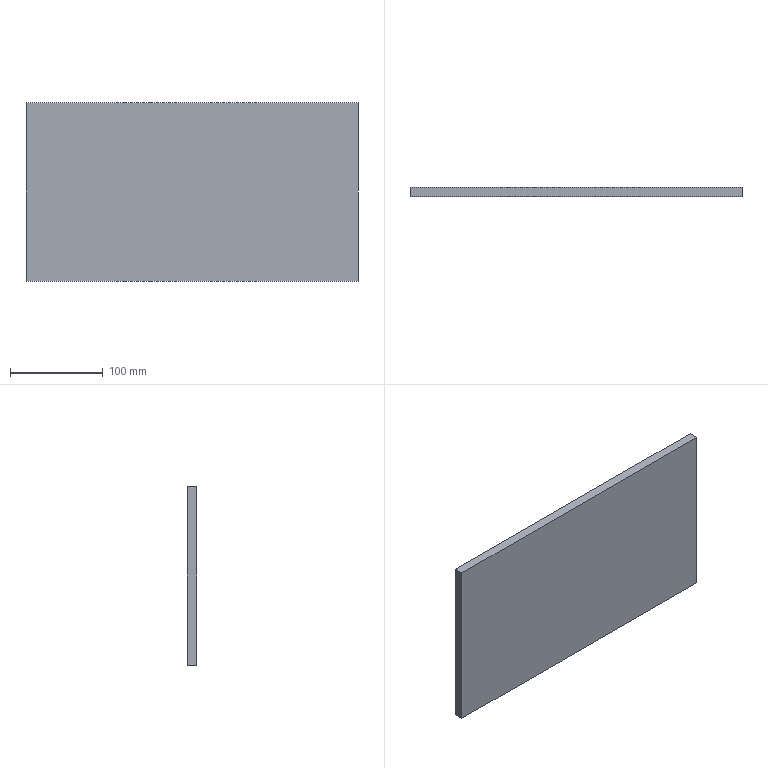Component | SolidWorks | ColumnRibPlate-1 | 1 solid | 6 faces | box 358 x 10 x 192 mm | volume 687360 mm3 | plane 6 | material Plain Carbon Steel
STEP:
#1=COLOUR_RGB('',0.7922,0.8196,0.9333);
#2=FILL_AREA_STYLE_COLOUR('',#1);
#3=FILL_AREA_STYLE('',(#2));
#4=SURFACE_STYLE_FILL_AREA(#3);
#5=SURFACE_SIDE_STYLE('',(#4));
#6=SURFACE_STYLE_USAGE(.BOTH.,#5);
#7=PRESENTATION_STYLE_ASSIGNMENT((#6));
#8=CARTESIAN_POINT('',(33.226,97.705,80.917));
#9=VERTEX_POINT('',#8);
#10=CARTESIAN_POINT('',(33.226,97.705,73.358));
#11=VERTEX_POINT('',#10);
#12=CARTESIAN_POINT('',(33.226,97.705,73.358));
#13=DIRECTION('',(-0.,0.,-1.));
#14=VECTOR('',#13,39.37);
#15=LINE('',#12,#14);
#16=EDGE_CURVE('',#9,#11,#15,.T.);
#17=ORIENTED_EDGE('',*,*,#16,.F.);
#18=CARTESIAN_POINT('',(33.226,97.311,80.917));
#19=VERTEX_POINT('',#18);
#20=CARTESIAN_POINT('',(33.226,97.311,80.917));
#21=DIRECTION('',(0.,1.,0.));
#22=VECTOR('',#21,39.37);
#23=LINE('',#20,#22);
#24=EDGE_CURVE('',#19,#9,#23,.T.);
#25=ORIENTED_EDGE('',*,*,#24,.F.);
#26=CARTESIAN_POINT('',(33.226,97.311,73.358));
#27=VERTEX_POINT('',#26);
#28=CARTESIAN_POINT('',(33.226,97.311,73.358));
#29=DIRECTION('',(-0.,0.,-1.));
#30=VECTOR('',#29,39.37);
#31=LINE('',#28,#30);
#32=EDGE_CURVE('',#19,#27,#31,.T.);
#33=ORIENTED_EDGE('',*,*,#32,.T.);
#34=CARTESIAN_POINT('',(33.226,97.311,73.358));
#35=DIRECTION('',(0.,1.,0.));
#36=VECTOR('',#35,39.37);
#37=LINE('',#34,#36);
#38=EDGE_CURVE('',#27,#11,#37,.T.);
#39=ORIENTED_EDGE('',*,*,#38,.T.);
#40=EDGE_LOOP('',(#17,#25,#33,#39));
#41=FACE_OUTER_BOUND('',#40,.T.);
#42=CARTESIAN_POINT('',(33.226,97.311,73.358));
#43=DIRECTION('',(1.,0.,-0.));
#44=DIRECTION('',(-0.,0.,-1.));
#45=AXIS2_PLACEMENT_3D('',#42,#43,#44);
#46=PLANE('',#45);
#47=ADVANCED_FACE('',(#41),#46,.T.);
#48=CARTESIAN_POINT('',(19.131,97.705,80.917));
#49=VERTEX_POINT('',#48);
#50=CARTESIAN_POINT('',(19.131,97.705,80.917));
#51=DIRECTION('',(1.,0.,0.));
#52=VECTOR('',#51,39.37);
#53=LINE('',#50,#52);
#54=EDGE_CURVE('',#49,#9,#53,.T.);
#55=ORIENTED_EDGE('',*,*,#54,.F.);
#56=CARTESIAN_POINT('',(19.131,97.311,80.917));
#57=VERTEX_POINT('',#56);
#58=CARTESIAN_POINT('',(19.131,97.311,80.917));
#59=DIRECTION('',(0.,1.,0.));
#60=VECTOR('',#59,39.37);
#61=LINE('',#58,#60);
#62=EDGE_CURVE('',#57,#49,#61,.T.);
#63=ORIENTED_EDGE('',*,*,#62,.F.);
#64=CARTESIAN_POINT('',(19.131,97.311,80.917));
#65=DIRECTION('',(1.,0.,0.));
#66=VECTOR('',#65,39.37);
#67=LINE('',#64,#66);
#68=EDGE_CURVE('',#57,#19,#67,.T.);
#69=ORIENTED_EDGE('',*,*,#68,.T.);
#70=ORIENTED_EDGE('',*,*,#24,.T.);
#71=EDGE_LOOP('',(#55,#63,#69,#70));
#72=FACE_OUTER_BOUND('',#71,.T.);
#73=CARTESIAN_POINT('',(19.131,97.311,80.917));
#74=DIRECTION('',(0.,0.,1.));
#75=DIRECTION('',(1.,0.,0.));
#76=AXIS2_PLACEMENT_3D('',#73,#74,#75);
#77=PLANE('',#76);
#78=ADVANCED_FACE('',(#72),#77,.T.);
#79=CARTESIAN_POINT('',(19.131,97.705,73.358));
#80=VERTEX_POINT('',#79);
#81=CARTESIAN_POINT('',(19.131,97.705,73.358));
#82=DIRECTION('',(0.,0.,1.));
#83=VECTOR('',#82,39.37);
#84=LINE('',#81,#83);
#85=EDGE_CURVE('',#80,#49,#84,.T.);
#86=ORIENTED_EDGE('',*,*,#85,.F.);
#87=CARTESIAN_POINT('',(19.131,97.311,73.358));
#88=VERTEX_POINT('',#87);
#89=CARTESIAN_POINT('',(19.131,97.311,73.358));
#90=DIRECTION('',(0.,1.,0.));
#91=VECTOR('',#90,39.37);
#92=LINE('',#89,#91);
#93=EDGE_CURVE('',#88,#80,#92,.T.);
#94=ORIENTED_EDGE('',*,*,#93,.F.);
#95=CARTESIAN_POINT('',(19.131,97.311,73.358));
#96=DIRECTION('',(0.,0.,1.));
#97=VECTOR('',#96,39.37);
#98=LINE('',#95,#97);
#99=EDGE_CURVE('',#88,#57,#98,.T.);
#100=ORIENTED_EDGE('',*,*,#99,.T.);
#101=ORIENTED_EDGE('',*,*,#62,.T.);
#102=EDGE_LOOP('',(#86,#94,#100,#101));
#103=FACE_OUTER_BOUND('',#102,.T.);
#104=CARTESIAN_POINT('',(19.131,97.311,73.358));
#105=DIRECTION('',(-1.,0.,0.));
#106=DIRECTION('',(0.,0.,1.));
#107=AXIS2_PLACEMENT_3D('',#104,#105,#106);
#108=PLANE('',#107);
#109=ADVANCED_FACE('',(#103),#108,.T.);
#110=CARTESIAN_POINT('',(19.131,97.705,73.358));
#111=DIRECTION('',(-1.,0.,0.));
#112=VECTOR('',#111,39.37);
#113=LINE('',#110,#112);
#114=EDGE_CURVE('',#11,#80,#113,.T.);
#115=ORIENTED_EDGE('',*,*,#114,.F.);
#116=ORIENTED_EDGE('',*,*,#38,.F.);
#117=CARTESIAN_POINT('',(19.131,97.311,73.358));
#118=DIRECTION('',(-1.,0.,0.));
#119=VECTOR('',#118,39.37);
#120=LINE('',#117,#119);
#121=EDGE_CURVE('',#27,#88,#120,.T.);
#122=ORIENTED_EDGE('',*,*,#121,.T.);
#123=ORIENTED_EDGE('',*,*,#93,.T.);
#124=EDGE_LOOP('',(#115,#116,#122,#123));
#125=FACE_OUTER_BOUND('',#124,.T.);
#126=CARTESIAN_POINT('',(19.131,97.311,73.358));
#127=DIRECTION('',(0.,0.,-1.));
#128=DIRECTION('',(-1.,0.,0.));
#129=AXIS2_PLACEMENT_3D('',#126,#127,#128);
#130=PLANE('',#129);
#131=ADVANCED_FACE('',(#125),#130,.T.);
#132=ORIENTED_EDGE('',*,*,#32,.F.);
#133=ORIENTED_EDGE('',*,*,#68,.F.);
#134=ORIENTED_EDGE('',*,*,#99,.F.);
#135=ORIENTED_EDGE('',*,*,#121,.F.);
#136=EDGE_LOOP('',(#132,#133,#134,#135));
#137=FACE_OUTER_BOUND('',#136,.T.);
#138=CARTESIAN_POINT('',(26.179,97.311,77.137));
#139=DIRECTION('',(0.,1.,0.));
#140=DIRECTION('',(0.,0.,1.));
#141=AXIS2_PLACEMENT_3D('',#138,#139,#140);
#142=PLANE('',#141);
#143=ADVANCED_FACE('',(#137),#142,.F.);
#144=ORIENTED_EDGE('',*,*,#16,.T.);
#145=ORIENTED_EDGE('',*,*,#114,.T.);
#146=ORIENTED_EDGE('',*,*,#85,.T.);
#147=ORIENTED_EDGE('',*,*,#54,.T.);
#148=EDGE_LOOP('',(#144,#145,#146,#147));
#149=FACE_OUTER_BOUND('',#148,.T.);
#150=CARTESIAN_POINT('',(26.179,97.705,77.137));
#151=DIRECTION('',(0.,1.,0.));
#152=DIRECTION('',(0.,0.,1.));
#153=AXIS2_PLACEMENT_3D('',#150,#151,#152);
#154=PLANE('',#153);
#155=ADVANCED_FACE('',(#149),#154,.T.);
#156=CLOSED_SHELL('',(#47,#78,#109,#131,#143,#155));
#157=MANIFOLD_SOLID_BREP('',#156);
#158=STYLED_ITEM('',(#7),#157);
#159=PRESENTATION_LAYER_ASSIGNMENT('','',(#158));
#160=CARTESIAN_POINT('',(0.,0.,0.));
#161=DIRECTION('',(0.,0.,1.));
#162=DIRECTION('',(1.,0.,0.));
#163=AXIS2_PLACEMENT_3D('',#160,#161,#162);
#164=(LENGTH_UNIT()NAMED_UNIT(*)SI_UNIT($,.METRE.));
#165=LENGTH_MEASURE_WITH_UNIT(LENGTH_MEASURE(0.0254),#164);
#166=DIMENSIONAL_EXPONENTS(1.,0.,0.,0.,0.,0.,0.);
#167=(CONVERSION_BASED_UNIT('',#165)LENGTH_UNIT()NAMED_UNIT(#166));
#168=UNCERTAINTY_MEASURE_WITH_UNIT(LENGTH_MEASURE(0.00001),#167,'','');
#169=(NAMED_UNIT(*)PLANE_ANGLE_UNIT()SI_UNIT($,.RADIAN.));
#170=(NAMED_UNIT(*)SI_UNIT($,.STERADIAN.)SOLID_ANGLE_UNIT());
#171=(GEOMETRIC_REPRESENTATION_CONTEXT(3)GLOBAL_UNCERTAINTY_ASSIGNED_CONTEXT((#168))GLOBAL_UNIT_ASSIGNED_CONTEXT((#167,#169,#170))REPRESENTATION_CONTEXT('',''));
#172=ADVANCED_BREP_SHAPE_REPRESENTATION('',(#157,#163),#171);
#173=(LENGTH_UNIT()NAMED_UNIT(*)SI_UNIT($,.METRE.));
#174=LENGTH_MEASURE_WITH_UNIT(LENGTH_MEASURE(0.0254),#173);
#175=DIMENSIONAL_EXPONENTS(1.,0.,0.,0.,0.,0.,0.);
#176=(CONVERSION_BASED_UNIT('',#174)LENGTH_UNIT()NAMED_UNIT(#175));
#177=UNCERTAINTY_MEASURE_WITH_UNIT(LENGTH_MEASURE(0.00001),#176,'','');
#178=(NAMED_UNIT(*)PLANE_ANGLE_UNIT()SI_UNIT($,.RADIAN.));
#179=(NAMED_UNIT(*)SI_UNIT($,.STERADIAN.)SOLID_ANGLE_UNIT());
#180=(GEOMETRIC_REPRESENTATION_CONTEXT(3)GLOBAL_UNCERTAINTY_ASSIGNED_CONTEXT((#177))GLOBAL_UNIT_ASSIGNED_CONTEXT((#176,#178,#179))REPRESENTATION_CONTEXT('',''));
#181=MECHANICAL_DESIGN_GEOMETRIC_PRESENTATION_REPRESENTATION('',(#158),#180);